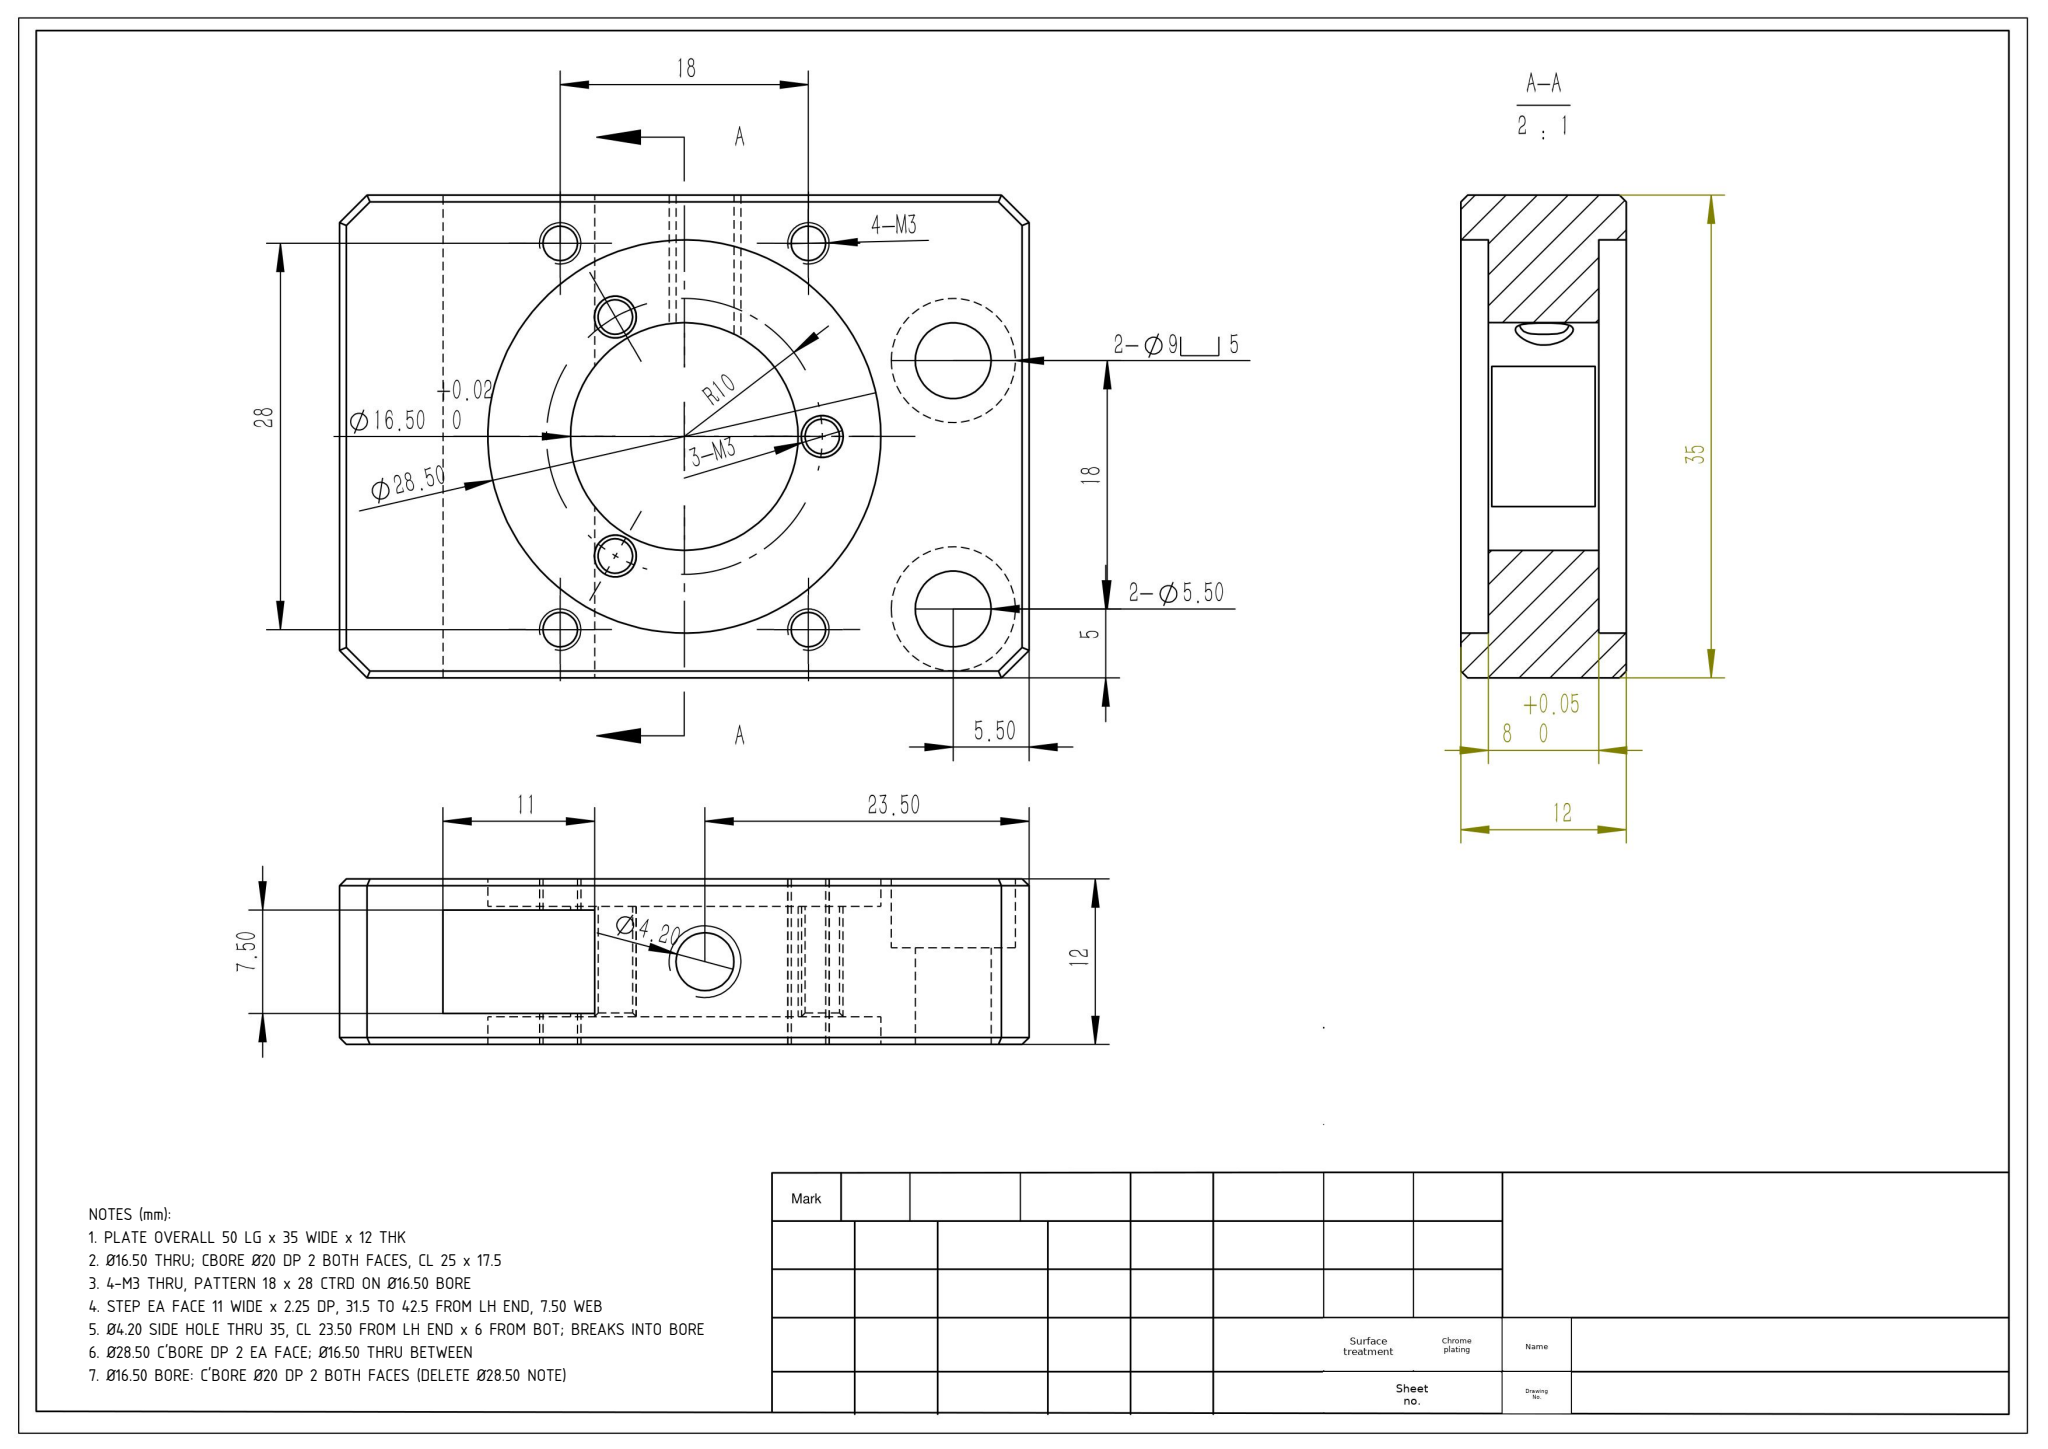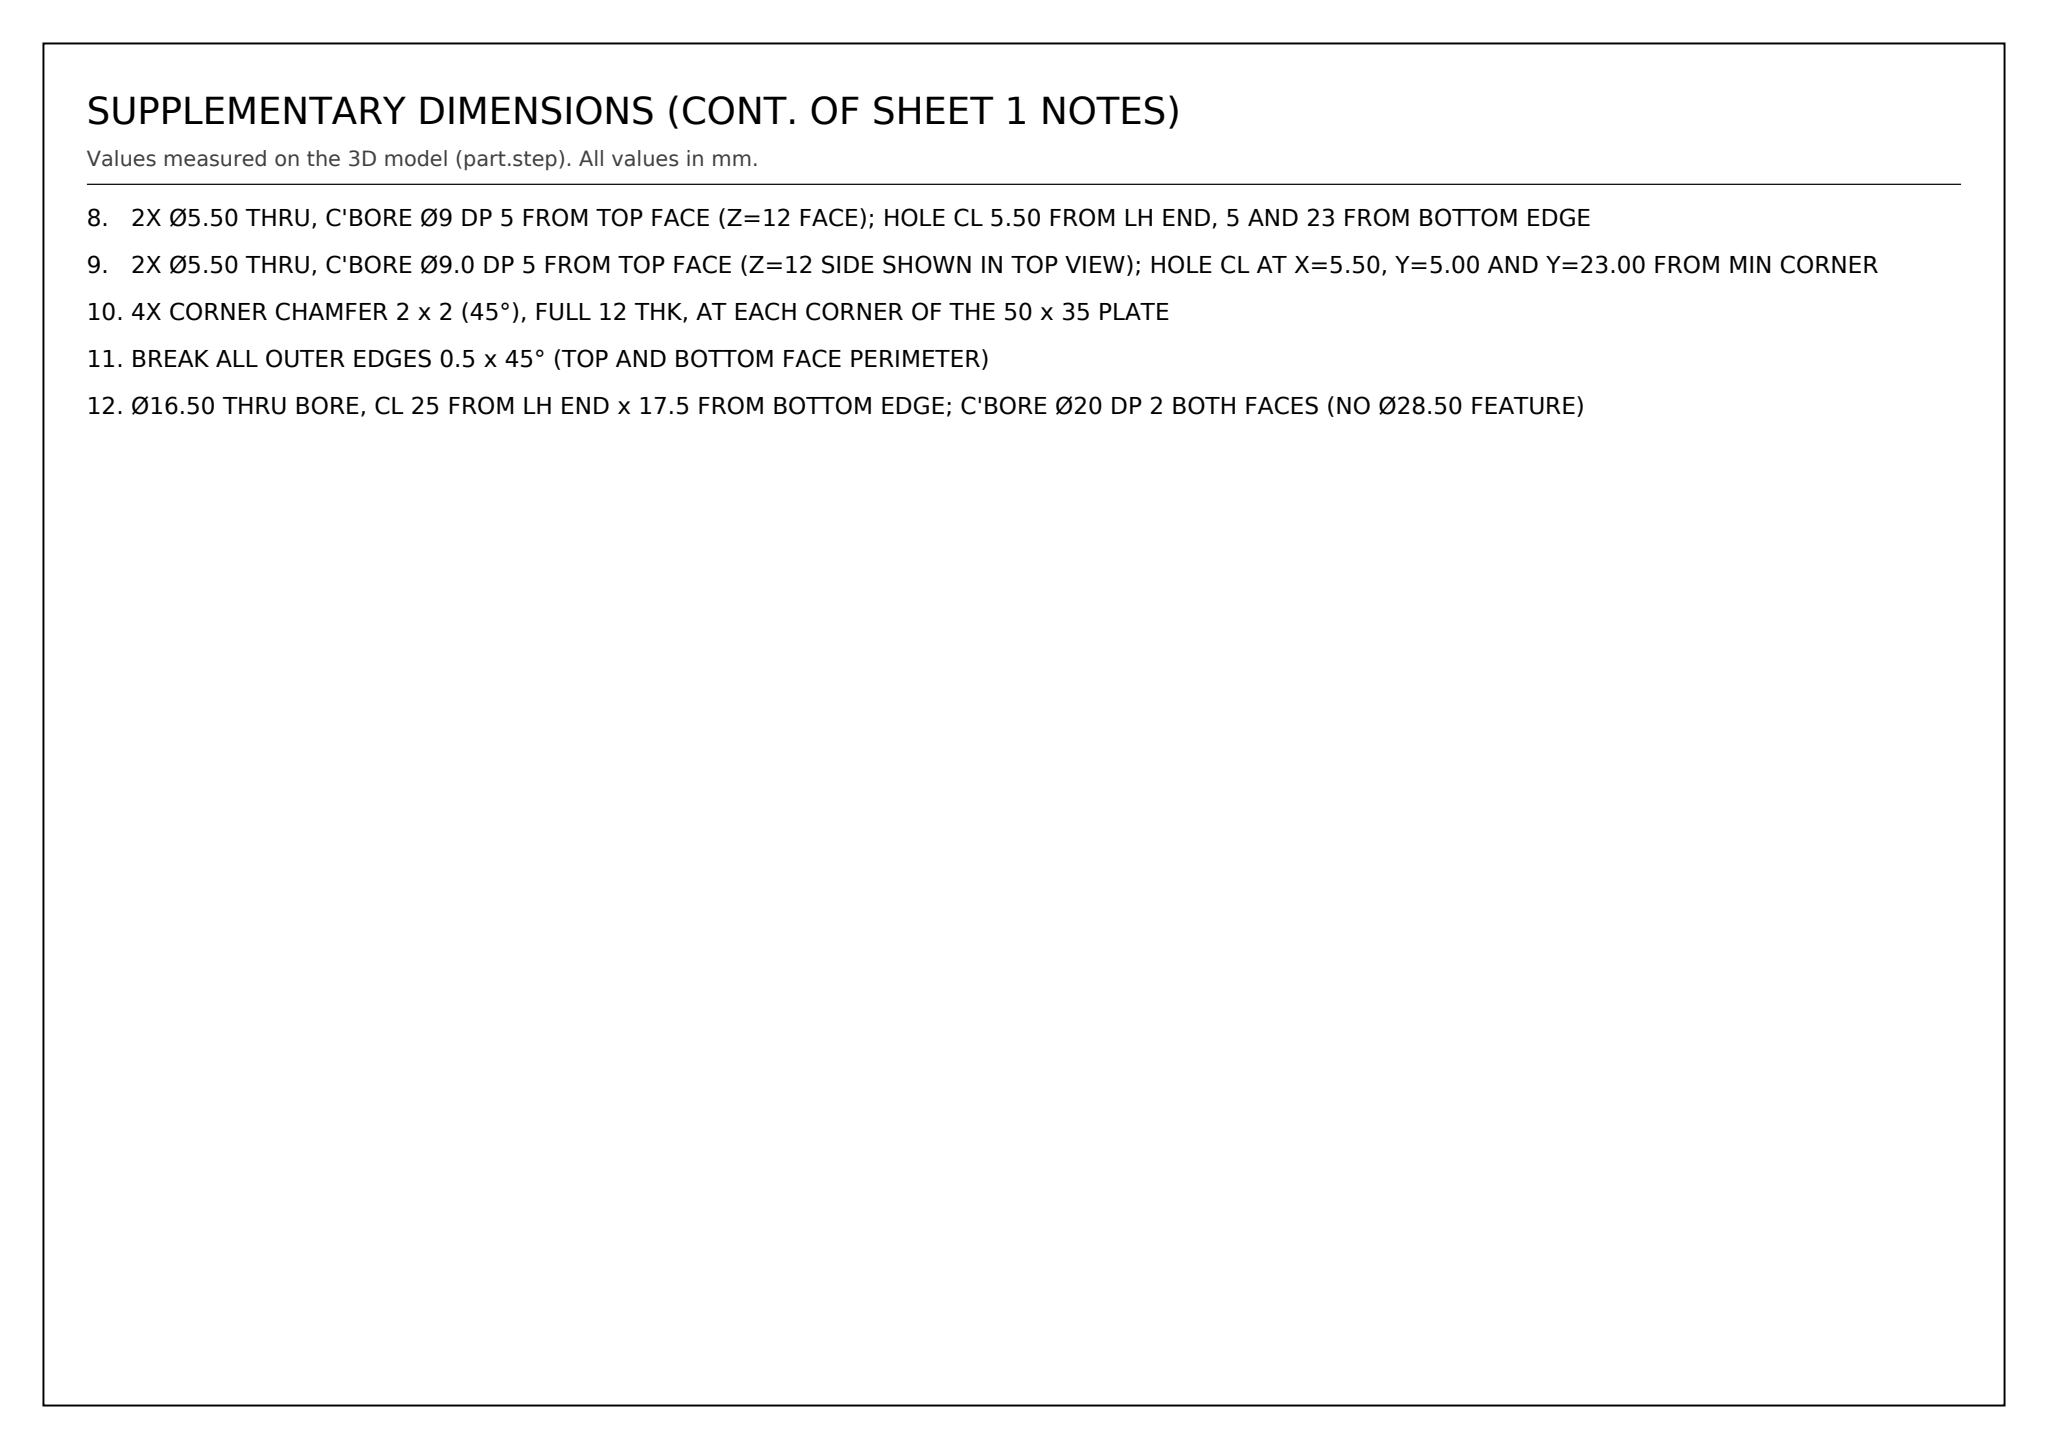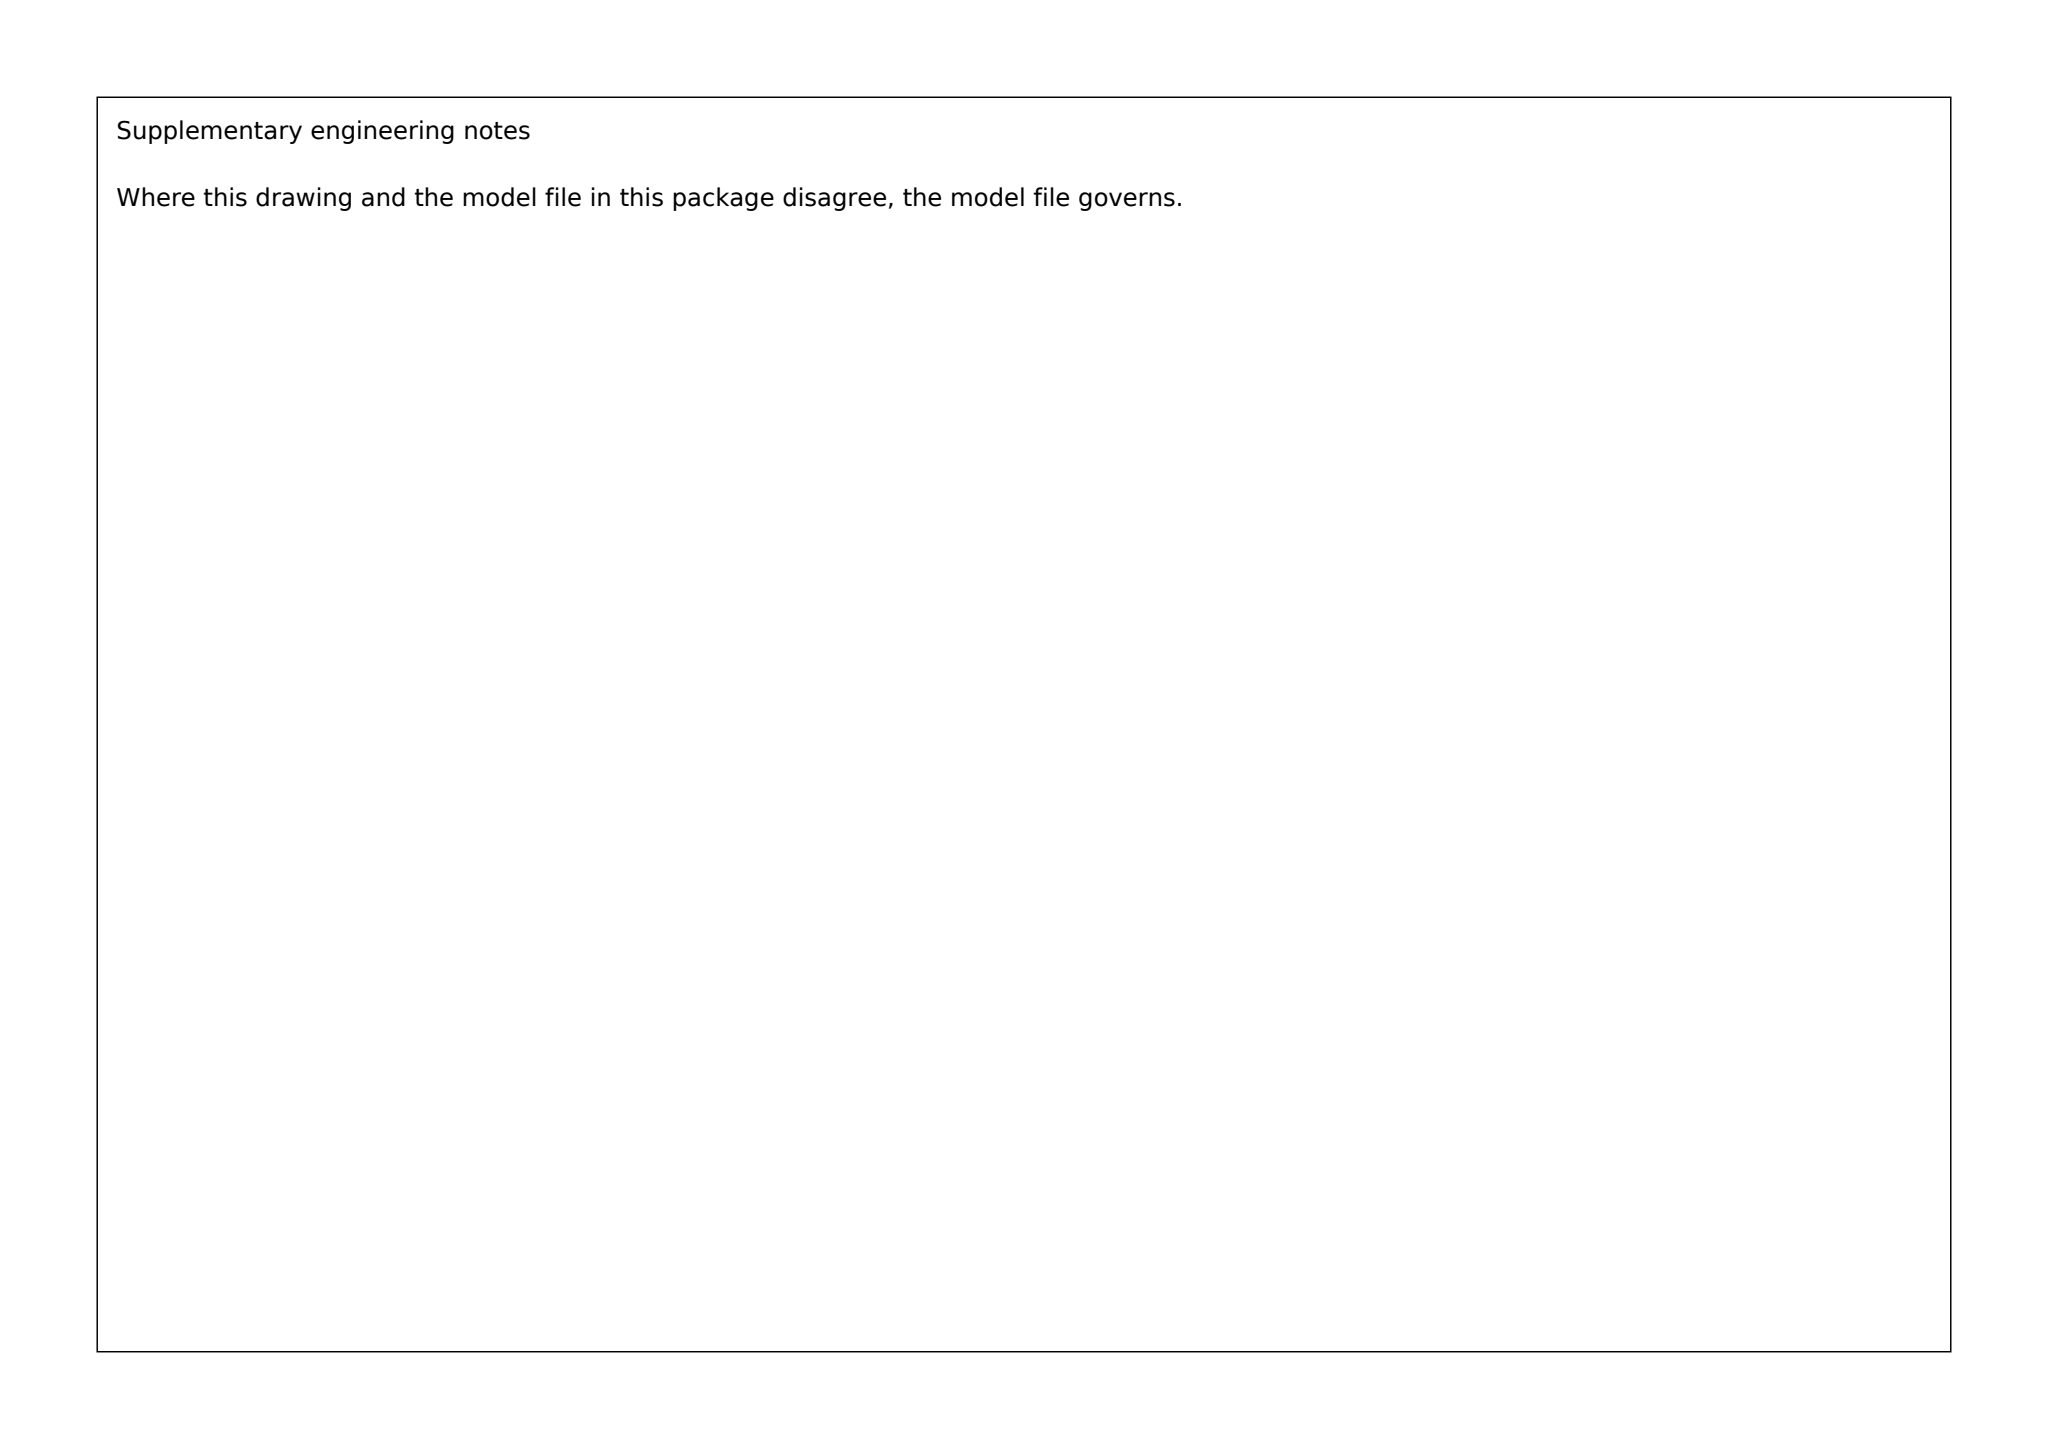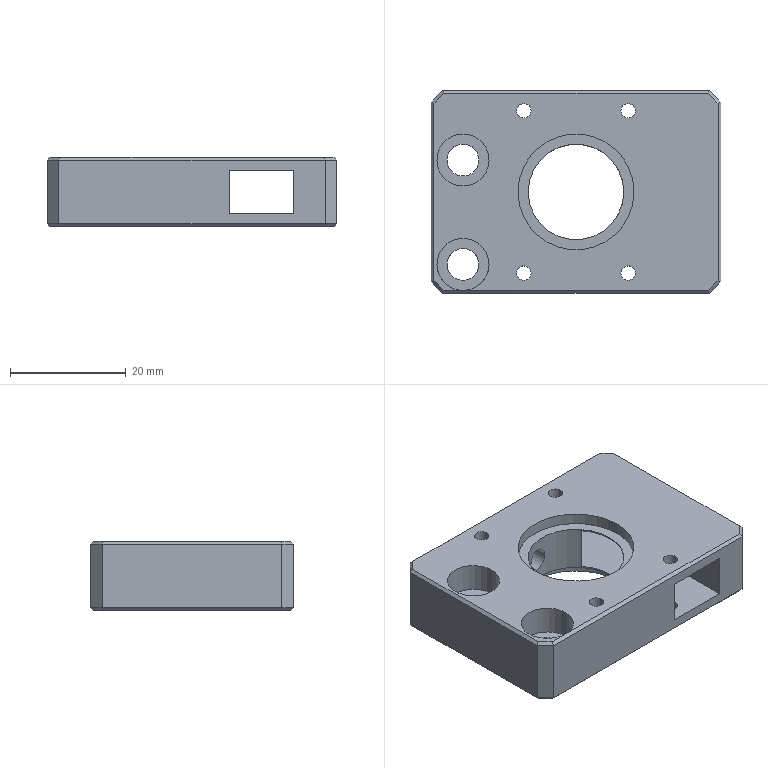Part | SolidWorks | mm | 1 solid | 63 faces | box 50 x 35 x 12 mm | volume 13837 mm3 | plane 35 | cylinder 28 | commonest cylinder face diameters 2.5 x12 9 x4 5.5 x4 20 x4 4.2 x2 16.5 x2
Drawing notes:
PLATE OVERALL 50 LG x 35 WIDE x 12 THK | from the solid: bbox_xyz = [50.0, 35.0, 12.0]
Ø16.50 THRU; CBORE Ø20 DP 2 BOTH FACES, CL 25 x 17.5 | from the solid: cyl Ø16.5 z-axis at (25,17.5) L=8.0; Ø20 same axis L=2.0 at z0-2 and z10-12
4-M3 THRU, PATTERN 18 x 28 CTRD ON Ø16.50 BORE | from the solid: Ø2.5 z-holes at x=16/34, y=3.5/31.5, L=12 thru; bore CL (25,17.5)
STEP EA FACE 11 WIDE x 2.25 DP, 31.5 TO 42.5 FROM LH END, 7.50 WEB | from the solid: x planes 31.5 & 42.5 (11 apart); z planes 2.25 & 9.75 = 2.25 dp ea face, 7.50 web
Ø4.20 SIDE HOLE THRU 35, CL 23.50 FROM LH END x 6 FROM BOT; BREAKS INTO BORE | from the solid: Ø4.2 y-axis cyl at x=23.5, z=6.0, segments 9.39 + 10.08 spanning 35, cut by Ø16.5 bore
Ø28.50 C'BORE DP 2 EA FACE; Ø16.50 THRU BETWEEN | from the solid: Counterbore cyls at bore axis (25,17.5): L=2.0 each face (z 0-2 and z 10-12, z-planes 2.0 & 10.0); Ø16.50 cyl L=8.0 spans z2-z10; STEP c'bore dia measures Ø20, drawing calls Ø28.50
Ø16.50 BORE: C'BORE Ø20 DP 2 BOTH FACES (DELETE Ø28.50 NOTE) | from the solid: cyl Ø20.0 axis z at (25.0,17.5), len 2.0, coaxial with Ø16.5 bore; z-planes at 2.0 and 10.0 give 2 deep from each 12 thk face
2X Ø5.50 THRU, C'BORE Ø9 DP 5 FROM TOP FACE (Z=12 FACE); HOLE CL 5.50 FROM LH END, 5 AND 23 FROM BOTTOM EDGE | from the solid: cylinders: Ø9.0 axis z at (5.5,5.0) and (5.5,23.0) length 5 starting at z-plane 7.0 up to z=12 top face; Ø5.5 axis z same XY, length 7 from z=0 to z=7 (total 12 = plate thickness)
2X Ø5.50 THRU, C'BORE Ø9.0 DP 5 FROM TOP FACE (Z=12 SIDE SHOWN IN TOP VIEW); HOLE CL AT X=5.50, Y=5.00 AND Y=23.00 FROM MIN CORNER | from the solid: cylinders [5.5,z,(5.5,5.0)/(5.5,23.0),len 7.0] and [9.0,z,same CL,len 5.0] with z-plane at 7.0 in 12 THK plate
4X CORNER CHAMFER 2 x 2 (45°), FULL 12 THK, AT EACH CORNER OF THE 50 x 35 PLATE | from the solid: inclined_planes angle_to_xyz [45,45,90], bbox_from [0,0,0.5] / [0,33,0.5] / [48,0,0.5] / [48,33,0.5], size [2,2,11]
BREAK ALL OUTER EDGES 0.5 x 45° (TOP AND BOTTOM FACE PERIMETER) | from the solid: inclined_planes angle_to_xyz [45,90,45] and [90,45,45], size 0.5 x 0.5 along the 50 and 35 edges at z=0 and z=11.5
Ø16.50 THRU BORE, CL 25 FROM LH END x 17.5 FROM BOTTOM EDGE; C'BORE Ø20 DP 2 BOTH FACES (NO Ø28.50 FEATURE) | from the solid: cylinders: dia 16.5 axis z at (25,17.5) from 2 to 10; dia 20 axis z at (25,17.5) from 0 to 2 and from 10 to 12
build123d program:
from build123d import *

# Parameters (mm, degrees)
SKETCH1_W                                           = 50
SKETCH1_H                                           = 35
BOSS_EXTRUDE1_DEPTH                                 = 6
CHAMFER1_SIZE                                       = 2
SKETCH4_R                                           = 8.25
CUT_EXTRUDE1_DEPTH                                  = 33.791
SKETCH5_R                                           = 10
CUT_EXTRUDE2_DEPTH                                  = 2
CUT_EXTRUDE3_START                                  = -2
SKETCH6_R                                           = 10
CUT_EXTRUDE3_DEPTH                                  = 2
SKETCH8_W                                           = 11
SKETCH8_H                                           = 7.5
CUT_EXTRUDE6_DEPTH                                  = 44.428
M3_TAPPED_HOLE2_D                                   = 2.5
M5_TAPPED_HOLE1_D                                   = 4.2
M5_TAPPED_HOLE1_DEPTH                               = 15
M5_TAPPED_HOLE1_TIP                                 = 1.262
CHAMFER2_SIZE                                       = 0.5
CYLINDRICAL_COUNTERSUNK_HOLE_FOR_M5_HEX_D           = 5.5
CYLINDRICAL_COUNTERSUNK_HOLE_FOR_M5_HEX_CBORE_D     = 9
CYLINDRICAL_COUNTERSUNK_HOLE_FOR_M5_HEX_CBORE_DEPTH = 5


with BuildPart() as part:
    # Sketch1 → Boss-Extrude1 (new, symmetric)
    with BuildSketch(Plane.XY):
        Rectangle(SKETCH1_W, SKETCH1_H)
    extrude(amount=BOSS_EXTRUDE1_DEPTH, both=True)

    # Chamfer1
    chamfer1_edges = [part.edges().sort_by_distance(p)[0] for p in [
        (25, -17.5, 0),
        (-25, -17.5, 0),
        (-25, 17.5, 0),
        (25, 17.5, 0),
    ]]
    chamfer(chamfer1_edges, length=CHAMFER1_SIZE)

    # Sketch4 → Cut-Extrude1 (cut, through all)
    with BuildSketch(Plane.XY.offset(6)):
        Circle(SKETCH4_R)
    extrude(amount=-CUT_EXTRUDE1_DEPTH, mode=Mode.SUBTRACT)

    # Sketch5 → Cut-Extrude2 (cut)
    with BuildSketch(Plane.XY.offset(6)):
        Circle(SKETCH5_R)
    extrude(amount=-CUT_EXTRUDE2_DEPTH, mode=Mode.SUBTRACT)

    # Sketch6 → Cut-Extrude3 (cut)
    with BuildSketch(Plane(origin=(0, 0, -6), x_dir=(-1, 0, 0), z_dir=(0, 0, -1)).offset(CUT_EXTRUDE3_START)):
        with Locations(Location((0, 0, 0), (0, 0, 180))):
            Circle(SKETCH6_R)
    extrude(amount=CUT_EXTRUDE3_DEPTH, mode=Mode.SUBTRACT)

    # Sketch8 → Cut-Extrude6 (cut, through all)
    with BuildSketch(Plane(origin=(0, 17.5, 0), x_dir=(1, 0, 0), z_dir=(0, 1, 0))):
        with Locations((12, 0)):
            Rectangle(SKETCH8_W, SKETCH8_H)
    extrude(amount=-CUT_EXTRUDE6_DEPTH, mode=Mode.SUBTRACT)

    # M3 Tapped Hole2 (through all)
    with Locations(Plane.XY.offset(6)):
        with Locations((-9, 14), (9, 14), (9, -14), (-9, -14)):
            Hole(M3_TAPPED_HOLE2_D / 2)

    # M5 Tapped Hole1
    with Locations(Plane(origin=(0, 17.5, 0), x_dir=(1, 0, 0), z_dir=(0, 1, 0))):
        with Locations((-1.5, 0)):
            Hole(M5_TAPPED_HOLE1_D / 2, depth=M5_TAPPED_HOLE1_DEPTH)
            with Locations((0, 0, -(M5_TAPPED_HOLE1_DEPTH + M5_TAPPED_HOLE1_TIP / 2))):  # 118° drill point
                Cone(0, M5_TAPPED_HOLE1_D / 2, M5_TAPPED_HOLE1_TIP, mode=Mode.SUBTRACT)

    # Chamfer2
    chamfer2_edges = [part.edges().sort_by_distance(p)[0] for p in [
        (0, 17.5, -6),
        (0, 17.5, 6),
        (25, 0, -6),
        (0, -17.5, -6),
        (-25, 0, -6),
        (-24, 16.5, -6),
        (-24, -16.5, -6),
        (24, -16.5, -6),
        (24, 16.5, -6),
        (25, 0, 6),
        (-25, 0, 6),
        (0, -17.5, 6),
        (-24, 16.5, 6),
        (-24, -16.5, 6),
        (24, -16.5, 6),
        (24, 16.5, 6),
    ]]
    chamfer(chamfer2_edges, length=CHAMFER2_SIZE)

    # Cylindrical Countersunk Hole for M5 Hex (through all)
    with Locations(Plane.XY.offset(6)):
        with Locations((-19.5, -12.5), (-19.5, 5.5)):
            CounterBoreHole(CYLINDRICAL_COUNTERSUNK_HOLE_FOR_M5_HEX_D / 2, CYLINDRICAL_COUNTERSUNK_HOLE_FOR_M5_HEX_CBORE_D / 2, CYLINDRICAL_COUNTERSUNK_HOLE_FOR_M5_HEX_CBORE_DEPTH)


solid = part.part